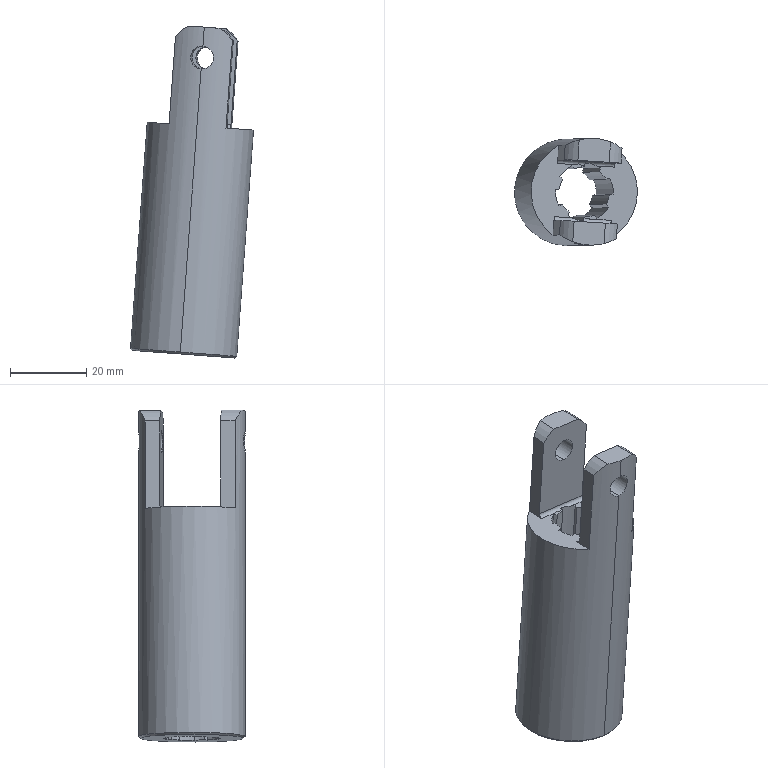Component | SolidWorks | UniversalJointC-1 | 1 solid | 54 faces | volume 30918 mm3 | cylinder 27 | plane 25 | cone 2 | commonest cylinder face diameters 15.2 x7 13.2 x6 6 x4 18 x4 28 x2 2 x2 15 x2